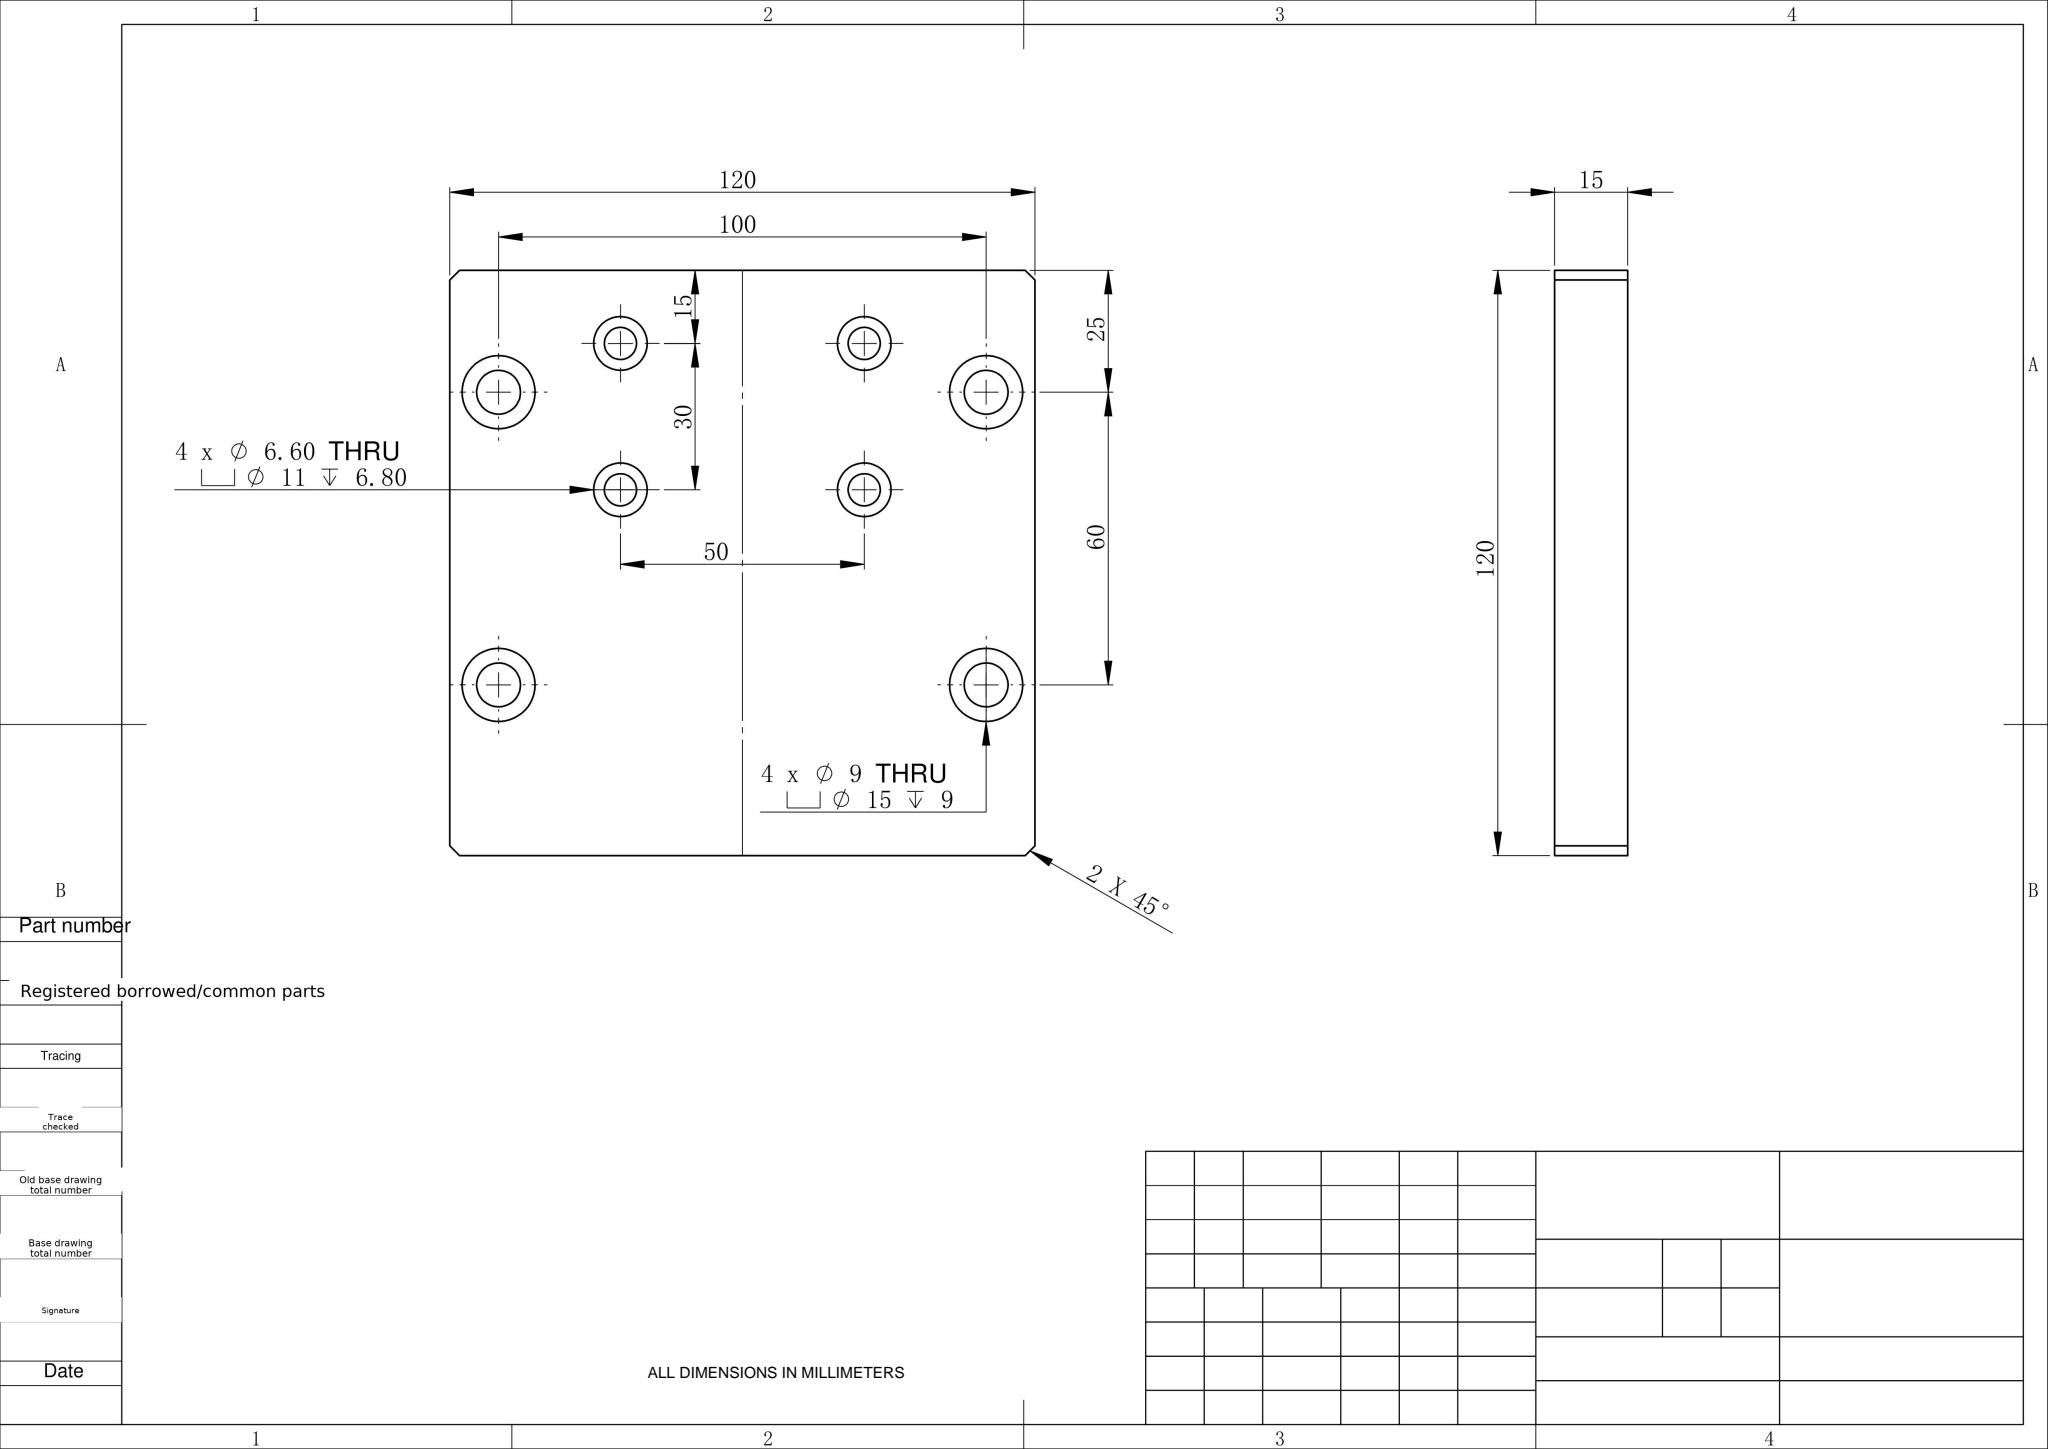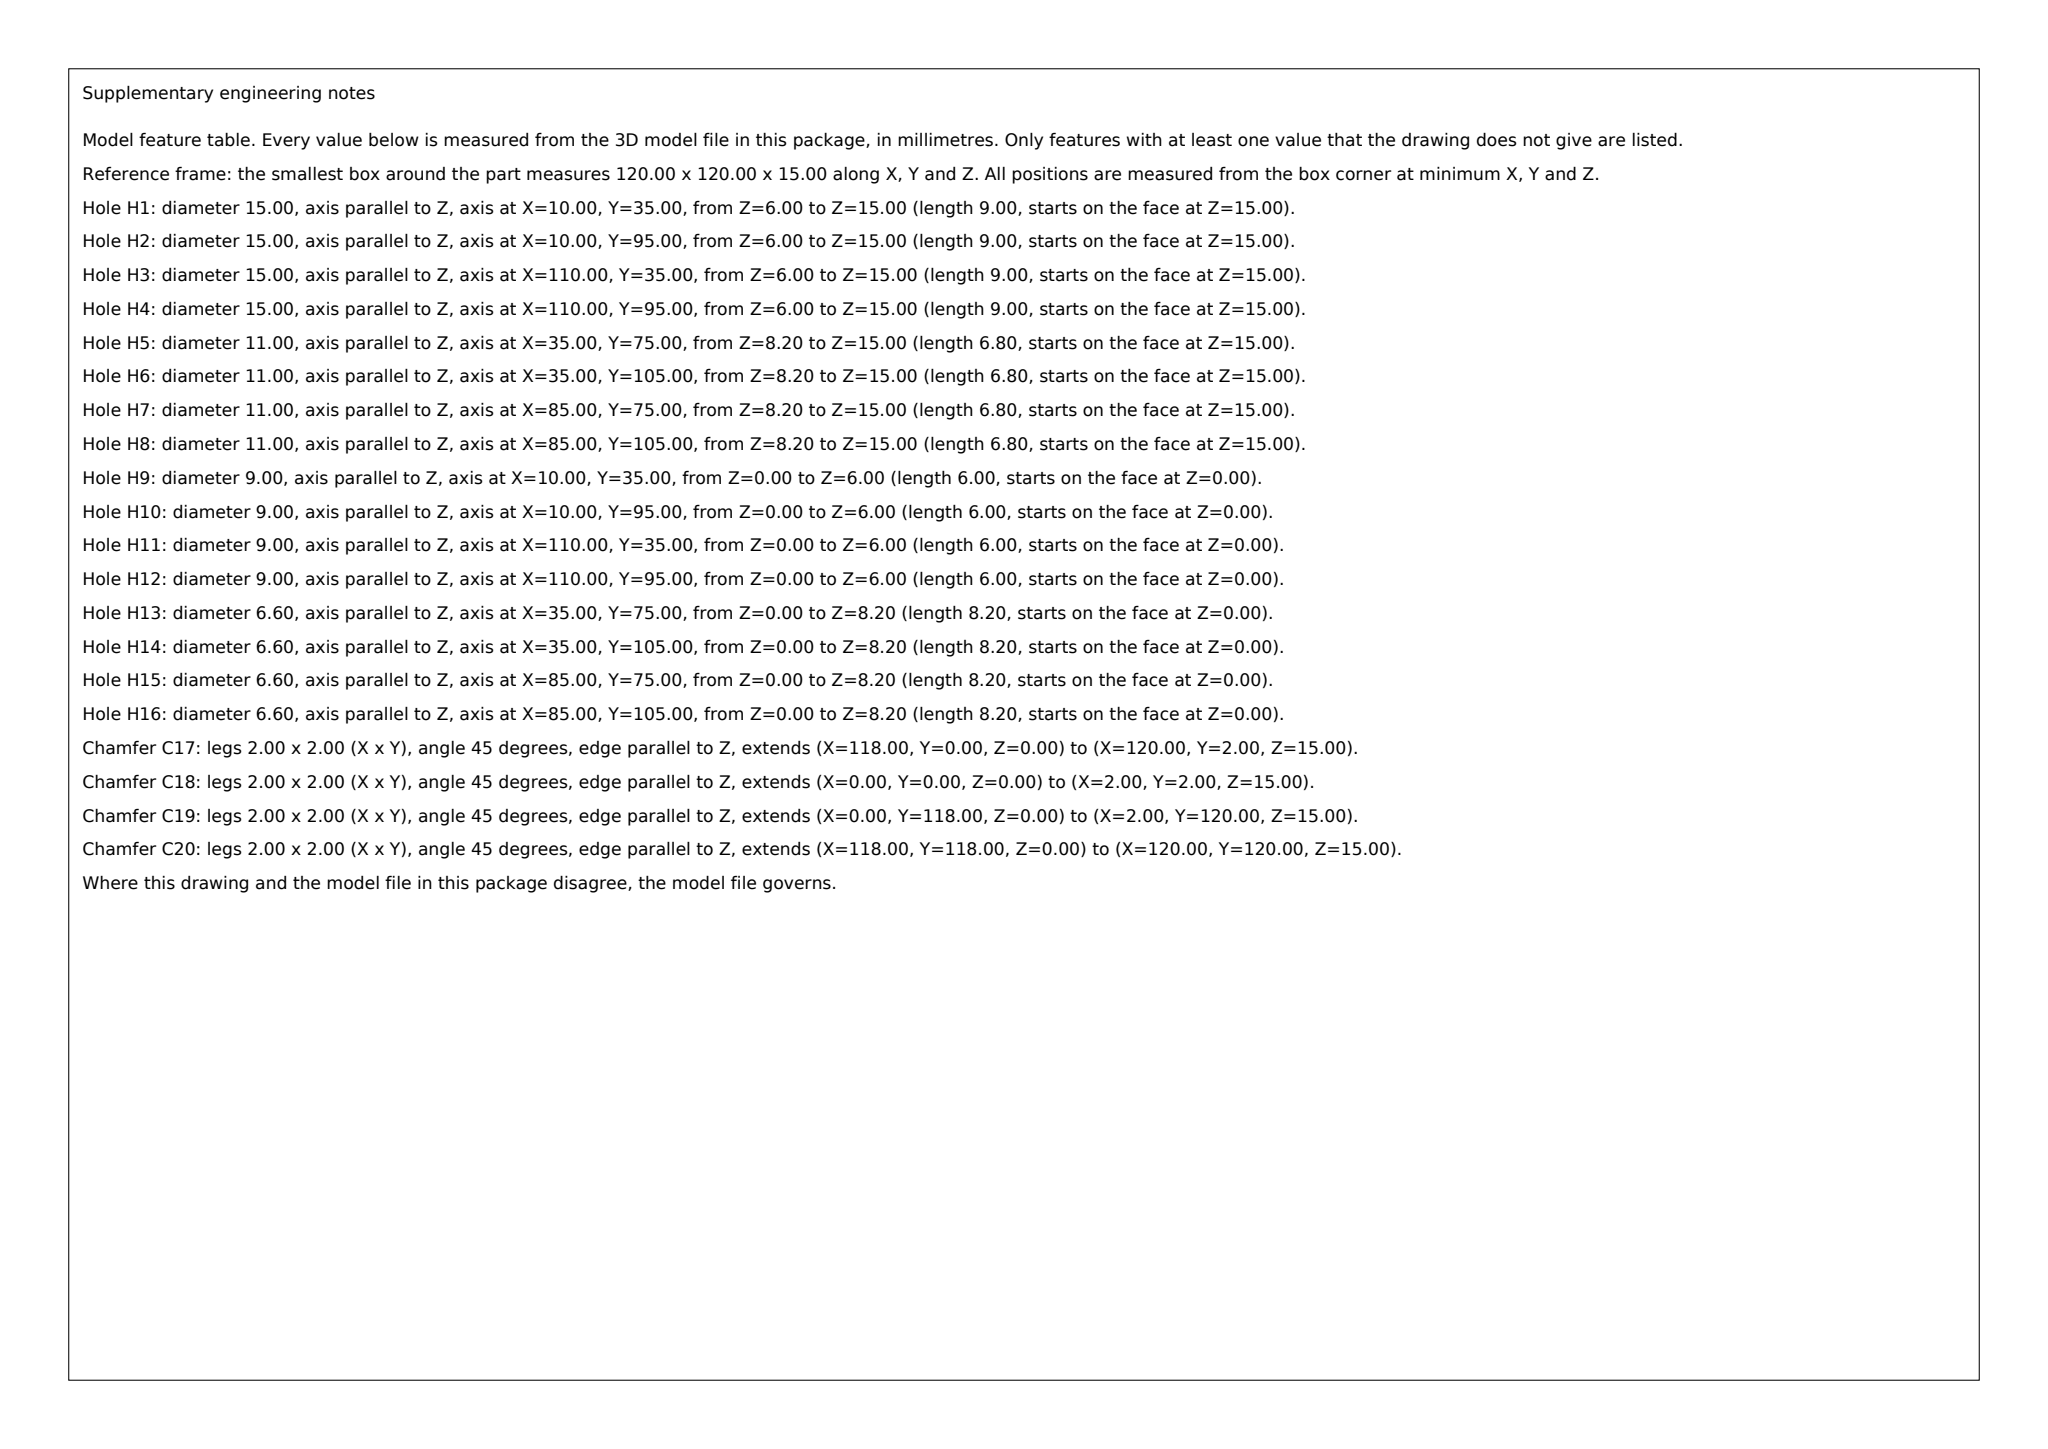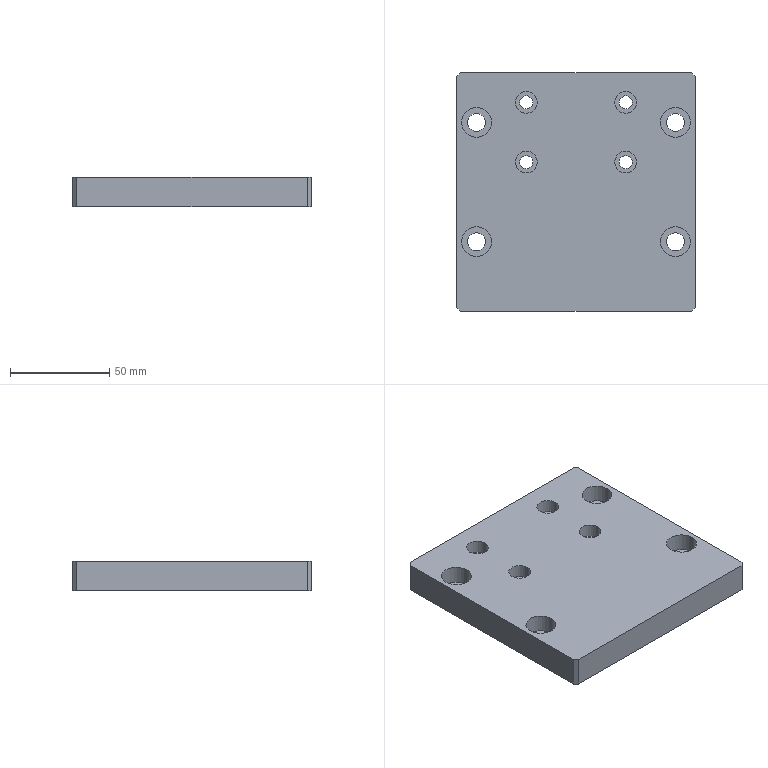Part | SolidWorks | mm | 1 solid | 50 faces | box 120 x 120 x 15 mm | volume 204284 mm3 | cylinder 32 | plane 18 | commonest cylinder face diameters 11 x8 6.6 x8 15 x8 9 x8
build123d program:
from build123d import *

# Parameters (mm, degrees)
SKETCH1_W                                         = 120
SKETCH1_H                                         = 120
BOSS_EXTRUDE1_DEPTH                               = 15
CHAMFER1_SIZE                                     = 2
HOLE_SIZE_ACCORDING_TO_HEXAGON_SOCKET_D           = 9
HOLE_SIZE_ACCORDING_TO_HEXAGON_SOCKET_CBORE_D     = 15
HOLE_SIZE_ACCORDING_TO_HEXAGON_SOCKET_CBORE_DEPTH = 9
HOLE_SIZE_ACCORDING_TO_HEXAGON_SO_2_D             = 6.6
HOLE_SIZE_ACCORDING_TO_HEXAGON_SO_2_CBORE_D       = 11
HOLE_SIZE_ACCORDING_TO_HEXAGON_SO_2_CBORE_DEPTH   = 6.8


with BuildPart() as part:
    # Sketch1 → Boss-Extrude1 (new body)
    with BuildSketch(Plane.XY):
        Rectangle(SKETCH1_W, SKETCH1_H)
    extrude(amount=BOSS_EXTRUDE1_DEPTH)

    # Chamfer1
    chamfer1_edges = [part.edges().sort_by_distance(p)[0] for p in [
        (-60, 60, 7.5),
        (60, 60, 7.5),
        (60, -60, 7.5),
        (-60, -60, 7.5),
    ]]
    chamfer(chamfer1_edges, length=CHAMFER1_SIZE)

    # Hole Size _ according to_ Hexagon Socket (through all)
    with Locations(Plane.XY.offset(15)):
        with Locations((50, -25), (-50, 35), (-50, -25), (50, 35)):
            CounterBoreHole(HOLE_SIZE_ACCORDING_TO_HEXAGON_SOCKET_D / 2, HOLE_SIZE_ACCORDING_TO_HEXAGON_SOCKET_CBORE_D / 2, HOLE_SIZE_ACCORDING_TO_HEXAGON_SOCKET_CBORE_DEPTH)

    # Hole Size _ according to_ Hexagon So 2 (through all)
    with Locations(Plane.XY.offset(15)):
        with Locations((-25, 45), (25, 15), (-25, 15), (25, 45)):
            CounterBoreHole(HOLE_SIZE_ACCORDING_TO_HEXAGON_SO_2_D / 2, HOLE_SIZE_ACCORDING_TO_HEXAGON_SO_2_CBORE_D / 2, HOLE_SIZE_ACCORDING_TO_HEXAGON_SO_2_CBORE_DEPTH)


solid = part.part